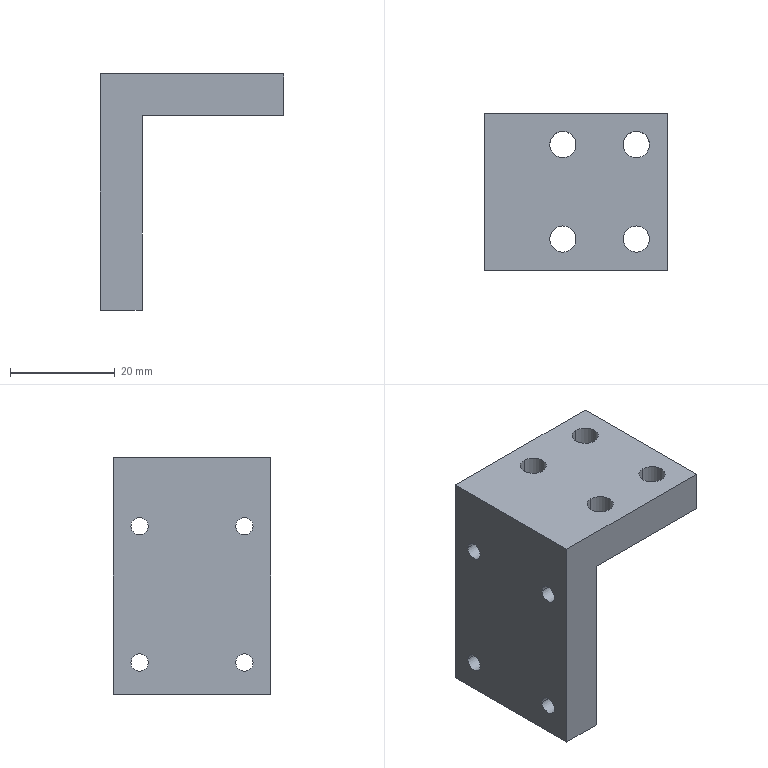Component | SolidWorks | DC-024-29-1 | 1 solid | 24 faces | box 35 x 30 x 45 mm | volume 16378 mm3 | cylinder 16 | plane 8 | commonest cylinder face diameters 3.3 x8 5 x8
build123d program:
from build123d import *

# Parameters (mm, degrees)
BOSS_EXTRUDE1_DEPTH = 15
M6_TAPPED_HOLE1_D   = 5
M4_TAPPED_HOLE1_D   = 3.3


with BuildPart() as part:
    # Sketch1 → Boss-Extrude1 (new, symmetric)
    with BuildSketch(Plane.XY):
        Polygon((-35, 0), (0, 0), (0, 45), (-8, 45), (-8, 8), (-35, 8), align=None)
    extrude(amount=BOSS_EXTRUDE1_DEPTH, both=True)

    # M6 Tapped Hole1 (through all)
    with Locations(Plane(origin=(0, 8, 0), x_dir=(1, 0, 0), z_dir=(0, 1, 0))):
        with Locations((-15, -9), (-15, 9), (-29, -9), (-29, 9)):
            Hole(M6_TAPPED_HOLE1_D / 2)

    # M4 Tapped Hole1 (through all)
    with Locations(Plane(origin=(0, 0, 0), x_dir=(0, 0, -1), z_dir=(1, 0, 0))):
        with Locations((10, 39), (-10, 39), (-10, 13), (10, 13)):
            Hole(M4_TAPPED_HOLE1_D / 2)


solid = part.part

# Placed as in the assembly
solid = solid.moved(Location((-61.333, 220.806, 63), (90, 0, -180)))
STEP:
#1=COLOUR_RGB('',0.7922,0.8196,0.9333);
#2=FILL_AREA_STYLE_COLOUR('',#1);
#3=FILL_AREA_STYLE('',(#2));
#4=SURFACE_STYLE_FILL_AREA(#3);
#5=SURFACE_SIDE_STYLE('',(#4));
#6=SURFACE_STYLE_USAGE(.BOTH.,#5);
#7=PRESENTATION_STYLE_ASSIGNMENT((#6));
#8=CARTESIAN_POINT('',(-2.1,9.022,0.9449));
#9=VERTEX_POINT('',#8);
#10=CARTESIAN_POINT('',(-2.1,9.152,0.9449));
#11=VERTEX_POINT('',#10);
#12=CARTESIAN_POINT('',(-2.1,9.087,0.9449));
#13=DIRECTION('',(-1.,0.,-0.));
#14=DIRECTION('',(0.,1.,0.));
#15=AXIS2_PLACEMENT_3D('',#12,#13,#14);
#16=CIRCLE('',#15,0.06496);
#17=EDGE_CURVE('',#9,#11,#16,.T.);
#18=ORIENTED_EDGE('',*,*,#17,.F.);
#19=CARTESIAN_POINT('',(-2.415,9.022,0.9449));
#20=VERTEX_POINT('',#19);
#21=CARTESIAN_POINT('',(-2.415,9.022,0.9449));
#22=DIRECTION('',(-1.,0.,-0.));
#23=VECTOR('',#22,39.37);
#24=LINE('',#21,#23);
#25=EDGE_CURVE('',#9,#20,#24,.T.);
#26=ORIENTED_EDGE('',*,*,#25,.T.);
#27=CARTESIAN_POINT('',(-2.415,9.152,0.9449));
#28=VERTEX_POINT('',#27);
#29=CARTESIAN_POINT('',(-2.415,9.087,0.9449));
#30=DIRECTION('',(-1.,0.,-0.));
#31=DIRECTION('',(0.,1.,0.));
#32=AXIS2_PLACEMENT_3D('',#29,#30,#31);
#33=CIRCLE('',#32,0.06496);
#34=EDGE_CURVE('',#20,#28,#33,.T.);
#35=ORIENTED_EDGE('',*,*,#34,.T.);
#36=CARTESIAN_POINT('',(-2.415,9.152,0.9449));
#37=DIRECTION('',(-1.,0.,-0.));
#38=VECTOR('',#37,39.37);
#39=LINE('',#36,#38);
#40=EDGE_CURVE('',#11,#28,#39,.T.);
#41=ORIENTED_EDGE('',*,*,#40,.F.);
#42=EDGE_LOOP('',(#18,#26,#35,#41));
#43=FACE_OUTER_BOUND('',#42,.T.);
#44=CARTESIAN_POINT('',(-2.415,9.087,0.9449));
#45=DIRECTION('',(-1.,0.,-0.));
#46=DIRECTION('',(0.,1.,0.));
#47=AXIS2_PLACEMENT_3D('',#44,#45,#46);
#48=CYLINDRICAL_SURFACE('',#47,0.06496);
#49=ADVANCED_FACE('',(#43),#48,.F.);
#50=CARTESIAN_POINT('',(-2.1,8.234,0.9449));
#51=VERTEX_POINT('',#50);
#52=CARTESIAN_POINT('',(-2.1,8.364,0.9449));
#53=VERTEX_POINT('',#52);
#54=CARTESIAN_POINT('',(-2.1,8.299,0.9449));
#55=DIRECTION('',(-1.,0.,-0.));
#56=DIRECTION('',(0.,1.,0.));
#57=AXIS2_PLACEMENT_3D('',#54,#55,#56);
#58=CIRCLE('',#57,0.06496);
#59=EDGE_CURVE('',#51,#53,#58,.T.);
#60=ORIENTED_EDGE('',*,*,#59,.F.);
#61=CARTESIAN_POINT('',(-2.415,8.234,0.9449));
#62=VERTEX_POINT('',#61);
#63=CARTESIAN_POINT('',(-2.415,8.234,0.9449));
#64=DIRECTION('',(-1.,0.,-0.));
#65=VECTOR('',#64,39.37);
#66=LINE('',#63,#65);
#67=EDGE_CURVE('',#51,#62,#66,.T.);
#68=ORIENTED_EDGE('',*,*,#67,.T.);
#69=CARTESIAN_POINT('',(-2.415,8.364,0.9449));
#70=VERTEX_POINT('',#69);
#71=CARTESIAN_POINT('',(-2.415,8.299,0.9449));
#72=DIRECTION('',(-1.,0.,-0.));
#73=DIRECTION('',(0.,1.,0.));
#74=AXIS2_PLACEMENT_3D('',#71,#72,#73);
#75=CIRCLE('',#74,0.06496);
#76=EDGE_CURVE('',#62,#70,#75,.T.);
#77=ORIENTED_EDGE('',*,*,#76,.T.);
#78=CARTESIAN_POINT('',(-2.415,8.364,0.9449));
#79=DIRECTION('',(-1.,0.,-0.));
#80=VECTOR('',#79,39.37);
#81=LINE('',#78,#80);
#82=EDGE_CURVE('',#53,#70,#81,.T.);
#83=ORIENTED_EDGE('',*,*,#82,.F.);
#84=EDGE_LOOP('',(#60,#68,#77,#83));
#85=FACE_OUTER_BOUND('',#84,.T.);
#86=CARTESIAN_POINT('',(-2.415,8.299,0.9449));
#87=DIRECTION('',(-1.,0.,-0.));
#88=DIRECTION('',(0.,1.,0.));
#89=AXIS2_PLACEMENT_3D('',#86,#87,#88);
#90=CYLINDRICAL_SURFACE('',#89,0.06496);
#91=ADVANCED_FACE('',(#85),#90,.F.);
#92=CARTESIAN_POINT('',(-2.1,8.234,1.969));
#93=VERTEX_POINT('',#92);
#94=CARTESIAN_POINT('',(-2.1,8.364,1.969));
#95=VERTEX_POINT('',#94);
#96=CARTESIAN_POINT('',(-2.1,8.299,1.969));
#97=DIRECTION('',(-1.,0.,-0.));
#98=DIRECTION('',(0.,1.,0.));
#99=AXIS2_PLACEMENT_3D('',#96,#97,#98);
#100=CIRCLE('',#99,0.06496);
#101=EDGE_CURVE('',#93,#95,#100,.T.);
#102=ORIENTED_EDGE('',*,*,#101,.F.);
#103=CARTESIAN_POINT('',(-2.415,8.234,1.969));
#104=VERTEX_POINT('',#103);
#105=CARTESIAN_POINT('',(-2.415,8.234,1.969));
#106=DIRECTION('',(-1.,0.,-0.));
#107=VECTOR('',#106,39.37);
#108=LINE('',#105,#107);
#109=EDGE_CURVE('',#93,#104,#108,.T.);
#110=ORIENTED_EDGE('',*,*,#109,.T.);
#111=CARTESIAN_POINT('',(-2.415,8.364,1.969));
#112=VERTEX_POINT('',#111);
#113=CARTESIAN_POINT('',(-2.415,8.299,1.969));
#114=DIRECTION('',(-1.,0.,-0.));
#115=DIRECTION('',(0.,1.,0.));
#116=AXIS2_PLACEMENT_3D('',#113,#114,#115);
#117=CIRCLE('',#116,0.06496);
#118=EDGE_CURVE('',#104,#112,#117,.T.);
#119=ORIENTED_EDGE('',*,*,#118,.T.);
#120=CARTESIAN_POINT('',(-2.415,8.364,1.969));
#121=DIRECTION('',(-1.,0.,-0.));
#122=VECTOR('',#121,39.37);
#123=LINE('',#120,#122);
#124=EDGE_CURVE('',#95,#112,#123,.T.);
#125=ORIENTED_EDGE('',*,*,#124,.F.);
#126=EDGE_LOOP('',(#102,#110,#119,#125));
#127=FACE_OUTER_BOUND('',#126,.T.);
#128=CARTESIAN_POINT('',(-2.415,8.299,1.969));
#129=DIRECTION('',(-1.,0.,-0.));
#130=DIRECTION('',(0.,1.,0.));
#131=AXIS2_PLACEMENT_3D('',#128,#129,#130);
#132=CYLINDRICAL_SURFACE('',#131,0.06496);
#133=ADVANCED_FACE('',(#127),#132,.F.);
#134=CARTESIAN_POINT('',(-2.1,9.022,1.969));
#135=VERTEX_POINT('',#134);
#136=CARTESIAN_POINT('',(-2.1,9.152,1.969));
#137=VERTEX_POINT('',#136);
#138=CARTESIAN_POINT('',(-2.1,9.087,1.969));
#139=DIRECTION('',(-1.,0.,-0.));
#140=DIRECTION('',(0.,1.,0.));
#141=AXIS2_PLACEMENT_3D('',#138,#139,#140);
#142=CIRCLE('',#141,0.06496);
#143=EDGE_CURVE('',#135,#137,#142,.T.);
#144=ORIENTED_EDGE('',*,*,#143,.F.);
#145=CARTESIAN_POINT('',(-2.415,9.022,1.969));
#146=VERTEX_POINT('',#145);
#147=CARTESIAN_POINT('',(-2.415,9.022,1.969));
#148=DIRECTION('',(-1.,0.,-0.));
#149=VECTOR('',#148,39.37);
#150=LINE('',#147,#149);
#151=EDGE_CURVE('',#135,#146,#150,.T.);
#152=ORIENTED_EDGE('',*,*,#151,.T.);
#153=CARTESIAN_POINT('',(-2.415,9.152,1.969));
#154=VERTEX_POINT('',#153);
#155=CARTESIAN_POINT('',(-2.415,9.087,1.969));
#156=DIRECTION('',(-1.,0.,-0.));
#157=DIRECTION('',(0.,1.,0.));
#158=AXIS2_PLACEMENT_3D('',#155,#156,#157);
#159=CIRCLE('',#158,0.06496);
#160=EDGE_CURVE('',#146,#154,#159,.T.);
#161=ORIENTED_EDGE('',*,*,#160,.T.);
#162=CARTESIAN_POINT('',(-2.415,9.152,1.969));
#163=DIRECTION('',(-1.,0.,-0.));
#164=VECTOR('',#163,39.37);
#165=LINE('',#162,#164);
#166=EDGE_CURVE('',#137,#154,#165,.T.);
#167=ORIENTED_EDGE('',*,*,#166,.F.);
#168=EDGE_LOOP('',(#144,#152,#161,#167));
#169=FACE_OUTER_BOUND('',#168,.T.);
#170=CARTESIAN_POINT('',(-2.415,9.087,1.969));
#171=DIRECTION('',(-1.,0.,-0.));
#172=DIRECTION('',(0.,1.,0.));
#173=AXIS2_PLACEMENT_3D('',#170,#171,#172);
#174=CYLINDRICAL_SURFACE('',#173,0.06496);
#175=ADVANCED_FACE('',(#169),#174,.F.);
#176=CARTESIAN_POINT('',(-1.824,8.437,2.48));
#177=VERTEX_POINT('',#176);
#178=CARTESIAN_POINT('',(-1.824,8.24,2.48));
#179=VERTEX_POINT('',#178);
#180=CARTESIAN_POINT('',(-1.824,8.339,2.48));
#181=DIRECTION('',(0.,-0.,-1.));
#182=DIRECTION('',(0.,-1.,0.));
#183=AXIS2_PLACEMENT_3D('',#180,#181,#182);
#184=CIRCLE('',#183,0.09843);
#185=EDGE_CURVE('',#177,#179,#184,.T.);
#186=ORIENTED_EDGE('',*,*,#185,.F.);
#187=CARTESIAN_POINT('',(-1.824,8.437,2.165));
#188=VERTEX_POINT('',#187);
#189=CARTESIAN_POINT('',(-1.824,8.437,2.165));
#190=DIRECTION('',(0.,-0.,-1.));
#191=VECTOR('',#190,39.37);
#192=LINE('',#189,#191);
#193=EDGE_CURVE('',#177,#188,#192,.T.);
#194=ORIENTED_EDGE('',*,*,#193,.T.);
#195=CARTESIAN_POINT('',(-1.824,8.24,2.165));
#196=VERTEX_POINT('',#195);
#197=CARTESIAN_POINT('',(-1.824,8.339,2.165));
#198=DIRECTION('',(0.,-0.,-1.));
#199=DIRECTION('',(0.,-1.,0.));
#200=AXIS2_PLACEMENT_3D('',#197,#198,#199);
#201=CIRCLE('',#200,0.09843);
#202=EDGE_CURVE('',#188,#196,#201,.T.);
#203=ORIENTED_EDGE('',*,*,#202,.T.);
#204=CARTESIAN_POINT('',(-1.824,8.24,2.165));
#205=DIRECTION('',(0.,-0.,-1.));
#206=VECTOR('',#205,39.37);
#207=LINE('',#204,#206);
#208=EDGE_CURVE('',#179,#196,#207,.T.);
#209=ORIENTED_EDGE('',*,*,#208,.F.);
#210=EDGE_LOOP('',(#186,#194,#203,#209));
#211=FACE_OUTER_BOUND('',#210,.T.);
#212=CARTESIAN_POINT('',(-1.824,8.339,2.165));
#213=DIRECTION('',(0.,-0.,-1.));
#214=DIRECTION('',(0.,-1.,0.));
#215=AXIS2_PLACEMENT_3D('',#212,#213,#214);
#216=CYLINDRICAL_SURFACE('',#215,0.09843);
#217=ADVANCED_FACE('',(#211),#216,.F.);
#218=CARTESIAN_POINT('',(-1.824,9.146,2.48));
#219=VERTEX_POINT('',#218);
#220=CARTESIAN_POINT('',(-1.824,8.949,2.48));
#221=VERTEX_POINT('',#220);
#222=CARTESIAN_POINT('',(-1.824,9.047,2.48));
#223=DIRECTION('',(0.,-0.,-1.));
#224=DIRECTION('',(0.,-1.,0.));
#225=AXIS2_PLACEMENT_3D('',#222,#223,#224);
#226=CIRCLE('',#225,0.09843);
#227=EDGE_CURVE('',#219,#221,#226,.T.);
#228=ORIENTED_EDGE('',*,*,#227,.F.);
#229=CARTESIAN_POINT('',(-1.824,9.146,2.165));
#230=VERTEX_POINT('',#229);
#231=CARTESIAN_POINT('',(-1.824,9.146,2.165));
#232=DIRECTION('',(0.,-0.,-1.));
#233=VECTOR('',#232,39.37);
#234=LINE('',#231,#233);
#235=EDGE_CURVE('',#219,#230,#234,.T.);
#236=ORIENTED_EDGE('',*,*,#235,.T.);
#237=CARTESIAN_POINT('',(-1.824,8.949,2.165));
#238=VERTEX_POINT('',#237);
#239=CARTESIAN_POINT('',(-1.824,9.047,2.165));
#240=DIRECTION('',(0.,-0.,-1.));
#241=DIRECTION('',(0.,-1.,0.));
#242=AXIS2_PLACEMENT_3D('',#239,#240,#241);
#243=CIRCLE('',#242,0.09843);
#244=EDGE_CURVE('',#230,#238,#243,.T.);
#245=ORIENTED_EDGE('',*,*,#244,.T.);
#246=CARTESIAN_POINT('',(-1.824,8.949,2.165));
#247=DIRECTION('',(0.,-0.,-1.));
#248=VECTOR('',#247,39.37);
#249=LINE('',#246,#248);
#250=EDGE_CURVE('',#221,#238,#249,.T.);
#251=ORIENTED_EDGE('',*,*,#250,.F.);
#252=EDGE_LOOP('',(#228,#236,#245,#251));
#253=FACE_OUTER_BOUND('',#252,.T.);
#254=CARTESIAN_POINT('',(-1.824,9.047,2.165));
#255=DIRECTION('',(0.,-0.,-1.));
#256=DIRECTION('',(0.,-1.,0.));
#257=AXIS2_PLACEMENT_3D('',#254,#255,#256);
#258=CYLINDRICAL_SURFACE('',#257,0.09843);
#259=ADVANCED_FACE('',(#253),#258,.F.);
#260=CARTESIAN_POINT('',(-1.273,8.437,2.48));
#261=VERTEX_POINT('',#260);
#262=CARTESIAN_POINT('',(-1.273,8.24,2.48));
#263=VERTEX_POINT('',#262);
#264=CARTESIAN_POINT('',(-1.273,8.339,2.48));
#265=DIRECTION('',(0.,-0.,-1.));
#266=DIRECTION('',(0.,-1.,0.));
#267=AXIS2_PLACEMENT_3D('',#264,#265,#266);
#268=CIRCLE('',#267,0.09843);
#269=EDGE_CURVE('',#261,#263,#268,.T.);
#270=ORIENTED_EDGE('',*,*,#269,.F.);
#271=CARTESIAN_POINT('',(-1.273,8.437,2.165));
#272=VERTEX_POINT('',#271);
#273=CARTESIAN_POINT('',(-1.273,8.437,2.165));
#274=DIRECTION('',(0.,-0.,-1.));
#275=VECTOR('',#274,39.37);
#276=LINE('',#273,#275);
#277=EDGE_CURVE('',#261,#272,#276,.T.);
#278=ORIENTED_EDGE('',*,*,#277,.T.);
#279=CARTESIAN_POINT('',(-1.273,8.24,2.165));
#280=VERTEX_POINT('',#279);
#281=CARTESIAN_POINT('',(-1.273,8.339,2.165));
#282=DIRECTION('',(0.,-0.,-1.));
#283=DIRECTION('',(0.,-1.,0.));
#284=AXIS2_PLACEMENT_3D('',#281,#282,#283);
#285=CIRCLE('',#284,0.09843);
#286=EDGE_CURVE('',#272,#280,#285,.T.);
#287=ORIENTED_EDGE('',*,*,#286,.T.);
#288=CARTESIAN_POINT('',(-1.273,8.24,2.165));
#289=DIRECTION('',(0.,-0.,-1.));
#290=VECTOR('',#289,39.37);
#291=LINE('',#288,#290);
#292=EDGE_CURVE('',#263,#280,#291,.T.);
#293=ORIENTED_EDGE('',*,*,#292,.F.);
#294=EDGE_LOOP('',(#270,#278,#287,#293));
#295=FACE_OUTER_BOUND('',#294,.T.);
#296=CARTESIAN_POINT('',(-1.273,8.339,2.165));
#297=DIRECTION('',(0.,-0.,-1.));
#298=DIRECTION('',(0.,-1.,0.));
#299=AXIS2_PLACEMENT_3D('',#296,#297,#298);
#300=CYLINDRICAL_SURFACE('',#299,0.09843);
#301=ADVANCED_FACE('',(#295),#300,.F.);
#302=CARTESIAN_POINT('',(-1.273,9.146,2.48));
#303=VERTEX_POINT('',#302);
#304=CARTESIAN_POINT('',(-1.273,8.949,2.48));
#305=VERTEX_POINT('',#304);
#306=CARTESIAN_POINT('',(-1.273,9.047,2.48));
#307=DIRECTION('',(0.,-0.,-1.));
#308=DIRECTION('',(0.,-1.,0.));
#309=AXIS2_PLACEMENT_3D('',#306,#307,#308);
#310=CIRCLE('',#309,0.09843);
#311=EDGE_CURVE('',#303,#305,#310,.T.);
#312=ORIENTED_EDGE('',*,*,#311,.F.);
#313=CARTESIAN_POINT('',(-1.273,9.146,2.165));
#314=VERTEX_POINT('',#313);
#315=CARTESIAN_POINT('',(-1.273,9.146,2.165));
#316=DIRECTION('',(0.,-0.,-1.));
#317=VECTOR('',#316,39.37);
#318=LINE('',#315,#317);
#319=EDGE_CURVE('',#303,#314,#318,.T.);
#320=ORIENTED_EDGE('',*,*,#319,.T.);
#321=CARTESIAN_POINT('',(-1.273,8.949,2.165));
#322=VERTEX_POINT('',#321);
#323=CARTESIAN_POINT('',(-1.273,9.047,2.165));
#324=DIRECTION('',(0.,-0.,-1.));
#325=DIRECTION('',(0.,-1.,0.));
#326=AXIS2_PLACEMENT_3D('',#323,#324,#325);
#327=CIRCLE('',#326,0.09843);
#328=EDGE_CURVE('',#314,#322,#327,.T.);
#329=ORIENTED_EDGE('',*,*,#328,.T.);
#330=CARTESIAN_POINT('',(-1.273,8.949,2.165));
#331=DIRECTION('',(0.,-0.,-1.));
#332=VECTOR('',#331,39.37);
#333=LINE('',#330,#332);
#334=EDGE_CURVE('',#305,#322,#333,.T.);
#335=ORIENTED_EDGE('',*,*,#334,.F.);
#336=EDGE_LOOP('',(#312,#320,#329,#335));
#337=FACE_OUTER_BOUND('',#336,.T.);
#338=CARTESIAN_POINT('',(-1.273,9.047,2.165));
#339=DIRECTION('',(0.,-0.,-1.));
#340=DIRECTION('',(0.,-1.,0.));
#341=AXIS2_PLACEMENT_3D('',#338,#339,#340);
#342=CYLINDRICAL_SURFACE('',#341,0.09843);
#343=ADVANCED_FACE('',(#337),#342,.F.);
#344=CARTESIAN_POINT('',(-1.037,9.284,2.165));
#345=VERTEX_POINT('',#344);
#346=CARTESIAN_POINT('',(-1.037,9.284,2.48));
#347=VERTEX_POINT('',#346);
#348=CARTESIAN_POINT('',(-1.037,9.284,2.165));
#349=DIRECTION('',(-0.,0.,1.));
#350=VECTOR('',#349,39.37);
#351=LINE('',#348,#350);
#352=EDGE_CURVE('',#345,#347,#351,.T.);
#353=ORIENTED_EDGE('',*,*,#352,.T.);
#354=CARTESIAN_POINT('',(-1.037,8.103,2.48));
#355=VERTEX_POINT('',#354);
#356=CARTESIAN_POINT('',(-1.037,8.103,2.48));
#357=DIRECTION('',(0.,1.,-0.));
#358=VECTOR('',#357,39.37);
#359=LINE('',#356,#358);
#360=EDGE_CURVE('',#355,#347,#359,.T.);
#361=ORIENTED_EDGE('',*,*,#360,.F.);
#362=CARTESIAN_POINT('',(-1.037,8.103,2.165));
#363=VERTEX_POINT('',#362);
#364=CARTESIAN_POINT('',(-1.037,8.103,2.165));
#365=DIRECTION('',(-0.,0.,1.));
#366=VECTOR('',#365,39.37);
#367=LINE('',#364,#366);
#368=EDGE_CURVE('',#363,#355,#367,.T.);
#369=ORIENTED_EDGE('',*,*,#368,.F.);
#370=CARTESIAN_POINT('',(-1.037,8.103,2.165));
#371=DIRECTION('',(0.,1.,-0.));
#372=VECTOR('',#371,39.37);
#373=LINE('',#370,#372);
#374=EDGE_CURVE('',#363,#345,#373,.T.);
#375=ORIENTED_EDGE('',*,*,#374,.T.);
#376=EDGE_LOOP('',(#353,#361,#369,#375));
#377=FACE_OUTER_BOUND('',#376,.T.);
#378=CARTESIAN_POINT('',(-1.037,8.103,2.165));
#379=DIRECTION('',(-1.,0.,-0.));
#380=DIRECTION('',(0.,1.,-0.));
#381=AXIS2_PLACEMENT_3D('',#378,#379,#380);
#382=PLANE('',#381);
#383=ADVANCED_FACE('',(#377),#382,.F.);
#384=CARTESIAN_POINT('',(-1.824,8.339,2.48));
#385=DIRECTION('',(0.,-0.,-1.));
#386=DIRECTION('',(0.,-1.,0.));
#387=AXIS2_PLACEMENT_3D('',#384,#385,#386);
#388=CIRCLE('',#387,0.09843);
#389=EDGE_CURVE('',#179,#177,#388,.T.);
#390=ORIENTED_EDGE('',*,*,#389,.T.);
#391=ORIENTED_EDGE('',*,*,#185,.T.);
#392=EDGE_LOOP('',(#390,#391));
#393=FACE_BOUND('',#392,.T.);
#394=CARTESIAN_POINT('',(-1.824,9.047,2.48));
#395=DIRECTION('',(0.,-0.,-1.));
#396=DIRECTION('',(0.,-1.,0.));
#397=AXIS2_PLACEMENT_3D('',#394,#395,#396);
#398=CIRCLE('',#397,0.09843);
#399=EDGE_CURVE('',#221,#219,#398,.T.);
#400=ORIENTED_EDGE('',*,*,#399,.T.);
#401=ORIENTED_EDGE('',*,*,#227,.T.);
#402=EDGE_LOOP('',(#400,#401));
#403=FACE_BOUND('',#402,.T.);
#404=CARTESIAN_POINT('',(-1.273,8.339,2.48));
#405=DIRECTION('',(0.,-0.,-1.));
#406=DIRECTION('',(0.,-1.,0.));
#407=AXIS2_PLACEMENT_3D('',#404,#405,#406);
#408=CIRCLE('',#407,0.09843);
#409=EDGE_CURVE('',#263,#261,#408,.T.);
#410=ORIENTED_EDGE('',*,*,#409,.T.);
#411=ORIENTED_EDGE('',*,*,#269,.T.);
#412=EDGE_LOOP('',(#410,#411));
#413=FACE_BOUND('',#412,.T.);
#414=CARTESIAN_POINT('',(-1.273,9.047,2.48));
#415=DIRECTION('',(0.,-0.,-1.));
#416=DIRECTION('',(0.,-1.,0.));
#417=AXIS2_PLACEMENT_3D('',#414,#415,#416);
#418=CIRCLE('',#417,0.09843);
#419=EDGE_CURVE('',#305,#303,#418,.T.);
#420=ORIENTED_EDGE('',*,*,#419,.T.);
#421=ORIENTED_EDGE('',*,*,#311,.T.);
#422=EDGE_LOOP('',(#420,#421));
#423=FACE_BOUND('',#422,.T.);
#424=CARTESIAN_POINT('',(-2.415,9.284,2.48));
#425=VERTEX_POINT('',#424);
#426=CARTESIAN_POINT('',(-1.037,9.284,2.48));
#427=DIRECTION('',(-1.,0.,-0.));
#428=VECTOR('',#427,39.37);
#429=LINE('',#426,#428);
#430=EDGE_CURVE('',#347,#425,#429,.T.);
#431=ORIENTED_EDGE('',*,*,#430,.T.);
#432=CARTESIAN_POINT('',(-2.415,8.103,2.48));
#433=VERTEX_POINT('',#432);
#434=CARTESIAN_POINT('',(-2.415,8.103,2.48));
#435=DIRECTION('',(0.,1.,-0.));
#436=VECTOR('',#435,39.37);
#437=LINE('',#434,#436);
#438=EDGE_CURVE('',#433,#425,#437,.T.);
#439=ORIENTED_EDGE('',*,*,#438,.F.);
#440=CARTESIAN_POINT('',(-1.037,8.103,2.48));
#441=DIRECTION('',(-1.,0.,-0.));
#442=VECTOR('',#441,39.37);
#443=LINE('',#440,#442);
#444=EDGE_CURVE('',#355,#433,#443,.T.);
#445=ORIENTED_EDGE('',*,*,#444,.F.);
#446=ORIENTED_EDGE('',*,*,#360,.T.);
#447=EDGE_LOOP('',(#431,#439,#445,#446));
#448=FACE_OUTER_BOUND('',#447,.T.);
#449=CARTESIAN_POINT('',(-1.037,8.103,2.48));
#450=DIRECTION('',(0.,-0.,-1.));
#451=DIRECTION('',(-0.,-1.,0.));
#452=AXIS2_PLACEMENT_3D('',#449,#450,#451);
#453=PLANE('',#452);
#454=ADVANCED_FACE('',(#393,#403,#413,#423,#448),#453,.F.);
#455=CARTESIAN_POINT('',(-2.415,9.087,0.9449));
#456=DIRECTION('',(-1.,0.,-0.));
#457=DIRECTION('',(0.,1.,0.));
#458=AXIS2_PLACEMENT_3D('',#455,#456,#457);
#459=CIRCLE('',#458,0.06496);
#460=EDGE_CURVE('',#28,#20,#459,.T.);
#461=ORIENTED_EDGE('',*,*,#460,.F.);
#462=ORIENTED_EDGE('',*,*,#34,.F.);
#463=EDGE_LOOP('',(#461,#462));
#464=FACE_BOUND('',#463,.T.);
#465=CARTESIAN_POINT('',(-2.415,8.299,0.9449));
#466=DIRECTION('',(-1.,0.,-0.));
#467=DIRECTION('',(0.,1.,0.));
#468=AXIS2_PLACEMENT_3D('',#465,#466,#467);
#469=CIRCLE('',#468,0.06496);
#470=EDGE_CURVE('',#70,#62,#469,.T.);
#471=ORIENTED_EDGE('',*,*,#470,.F.);
#472=ORIENTED_EDGE('',*,*,#76,.F.);
#473=EDGE_LOOP('',(#471,#472));
#474=FACE_BOUND('',#473,.T.);
#475=CARTESIAN_POINT('',(-2.415,8.299,1.969));
#476=DIRECTION('',(-1.,0.,-0.));
#477=DIRECTION('',(0.,1.,0.));
#478=AXIS2_PLACEMENT_3D('',#475,#476,#477);
#479=CIRCLE('',#478,0.06496);
#480=EDGE_CURVE('',#112,#104,#479,.T.);
#481=ORIENTED_EDGE('',*,*,#480,.F.);
#482=ORIENTED_EDGE('',*,*,#118,.F.);
#483=EDGE_LOOP('',(#481,#482));
#484=FACE_BOUND('',#483,.T.);
#485=CARTESIAN_POINT('',(-2.415,9.087,1.969));
#486=DIRECTION('',(-1.,0.,-0.));
#487=DIRECTION('',(0.,1.,0.));
#488=AXIS2_PLACEMENT_3D('',#485,#486,#487);
#489=CIRCLE('',#488,0.06496);
#490=EDGE_CURVE('',#154,#146,#489,.T.);
#491=ORIENTED_EDGE('',*,*,#490,.F.);
#492=ORIENTED_EDGE('',*,*,#160,.F.);
#493=EDGE_LOOP('',(#491,#492));
#494=FACE_BOUND('',#493,.T.);
#495=CARTESIAN_POINT('',(-2.415,9.284,0.7087));
#496=VERTEX_POINT('',#495);
#497=CARTESIAN_POINT('',(-2.415,9.284,2.48));
#498=DIRECTION('',(0.,-0.,-1.));
#499=VECTOR('',#498,39.37);
#500=LINE('',#497,#499);
#501=EDGE_CURVE('',#425,#496,#500,.T.);
#502=ORIENTED_EDGE('',*,*,#501,.T.);
#503=CARTESIAN_POINT('',(-2.415,8.103,0.7087));
#504=VERTEX_POINT('',#503);
#505=CARTESIAN_POINT('',(-2.415,8.103,0.7087));
#506=DIRECTION('',(0.,1.,-0.));
#507=VECTOR('',#506,39.37);
#508=LINE('',#505,#507);
#509=EDGE_CURVE('',#504,#496,#508,.T.);
#510=ORIENTED_EDGE('',*,*,#509,.F.);
#511=CARTESIAN_POINT('',(-2.415,8.103,2.48));
#512=DIRECTION('',(0.,-0.,-1.));
#513=VECTOR('',#512,39.37);
#514=LINE('',#511,#513);
#515=EDGE_CURVE('',#433,#504,#514,.T.);
#516=ORIENTED_EDGE('',*,*,#515,.F.);
#517=ORIENTED_EDGE('',*,*,#438,.T.);
#518=EDGE_LOOP('',(#502,#510,#516,#517));
#519=FACE_OUTER_BOUND('',#518,.T.);
#520=CARTESIAN_POINT('',(-2.415,8.103,2.48));
#521=DIRECTION('',(1.,-0.,0.));
#522=DIRECTION('',(-0.,-1.,0.));
#523=AXIS2_PLACEMENT_3D('',#520,#521,#522);
#524=PLANE('',#523);
#525=ADVANCED_FACE('',(#464,#474,#484,#494,#519),#524,.F.);
#526=CARTESIAN_POINT('',(-2.1,9.284,0.7087));
#527=VERTEX_POINT('',#526);
#528=CARTESIAN_POINT('',(-2.1,9.284,0.7087));
#529=DIRECTION('',(1.,-0.,0.));
#530=VECTOR('',#529,39.37);
#531=LINE('',#528,#530);
#532=EDGE_CURVE('',#496,#527,#531,.T.);
#533=ORIENTED_EDGE('',*,*,#532,.T.);
#534=CARTESIAN_POINT('',(-2.1,8.103,0.7087));
#535=VERTEX_POINT('',#534);
#536=CARTESIAN_POINT('',(-2.1,8.103,0.7087));
#537=DIRECTION('',(0.,1.,-0.));
#538=VECTOR('',#537,39.37);
#539=LINE('',#536,#538);
#540=EDGE_CURVE('',#535,#527,#539,.T.);
#541=ORIENTED_EDGE('',*,*,#540,.F.);
#542=CARTESIAN_POINT('',(-2.1,8.103,0.7087));
#543=DIRECTION('',(1.,-0.,0.));
#544=VECTOR('',#543,39.37);
#545=LINE('',#542,#544);
#546=EDGE_CURVE('',#504,#535,#545,.T.);
#547=ORIENTED_EDGE('',*,*,#546,.F.);
#548=ORIENTED_EDGE('',*,*,#509,.T.);
#549=EDGE_LOOP('',(#533,#541,#547,#548));
#550=FACE_OUTER_BOUND('',#549,.T.);
#551=CARTESIAN_POINT('',(-2.1,8.103,0.7087));
#552=DIRECTION('',(-0.,0.,1.));
#553=DIRECTION('',(0.,1.,-0.));
#554=AXIS2_PLACEMENT_3D('',#551,#552,#553);
#555=PLANE('',#554);
#556=ADVANCED_FACE('',(#550),#555,.F.);
#557=CARTESIAN_POINT('',(-2.1,9.087,0.9449));
#558=DIRECTION('',(-1.,0.,-0.));
#559=DIRECTION('',(0.,1.,0.));
#560=AXIS2_PLACEMENT_3D('',#557,#558,#559);
#561=CIRCLE('',#560,0.06496);
#562=EDGE_CURVE('',#11,#9,#561,.T.);
#563=ORIENTED_EDGE('',*,*,#562,.T.);
#564=ORIENTED_EDGE('',*,*,#17,.T.);
#565=EDGE_LOOP('',(#563,#564));
#566=FACE_BOUND('',#565,.T.);
#567=CARTESIAN_POINT('',(-2.1,8.299,0.9449));
#568=DIRECTION('',(-1.,0.,-0.));
#569=DIRECTION('',(0.,1.,0.));
#570=AXIS2_PLACEMENT_3D('',#567,#568,#569);
#571=CIRCLE('',#570,0.06496);
#572=EDGE_CURVE('',#53,#51,#571,.T.);
#573=ORIENTED_EDGE('',*,*,#572,.T.);
#574=ORIENTED_EDGE('',*,*,#59,.T.);
#575=EDGE_LOOP('',(#573,#574));
#576=FACE_BOUND('',#575,.T.);
#577=CARTESIAN_POINT('',(-2.1,8.299,1.969));
#578=DIRECTION('',(-1.,0.,-0.));
#579=DIRECTION('',(0.,1.,0.));
#580=AXIS2_PLACEMENT_3D('',#577,#578,#579);
#581=CIRCLE('',#580,0.06496);
#582=EDGE_CURVE('',#95,#93,#581,.T.);
#583=ORIENTED_EDGE('',*,*,#582,.T.);
#584=ORIENTED_EDGE('',*,*,#101,.T.);
#585=EDGE_LOOP('',(#583,#584));
#586=FACE_BOUND('',#585,.T.);
#587=CARTESIAN_POINT('',(-2.1,9.087,1.969));
#588=DIRECTION('',(-1.,0.,-0.));
#589=DIRECTION('',(0.,1.,0.));
#590=AXIS2_PLACEMENT_3D('',#587,#588,#589);
#591=CIRCLE('',#590,0.06496);
#592=EDGE_CURVE('',#137,#135,#591,.T.);
#593=ORIENTED_EDGE('',*,*,#592,.T.);
#594=ORIENTED_EDGE('',*,*,#143,.T.);
#595=EDGE_LOOP('',(#593,#594));
#596=FACE_BOUND('',#595,.T.);
#597=CARTESIAN_POINT('',(-2.1,9.284,2.165));
#598=VERTEX_POINT('',#597);
#599=CARTESIAN_POINT('',(-2.1,9.284,2.165));
#600=DIRECTION('',(-0.,0.,1.));
#601=VECTOR('',#600,39.37);
#602=LINE('',#599,#601);
#603=EDGE_CURVE('',#527,#598,#602,.T.);
#604=ORIENTED_EDGE('',*,*,#603,.T.);
#605=CARTESIAN_POINT('',(-2.1,8.103,2.165));
#606=VERTEX_POINT('',#605);
#607=CARTESIAN_POINT('',(-2.1,8.103,2.165));
#608=DIRECTION('',(0.,1.,-0.));
#609=VECTOR('',#608,39.37);
#610=LINE('',#607,#609);
#611=EDGE_CURVE('',#606,#598,#610,.T.);
#612=ORIENTED_EDGE('',*,*,#611,.F.);
#613=CARTESIAN_POINT('',(-2.1,8.103,2.165));
#614=DIRECTION('',(-0.,0.,1.));
#615=VECTOR('',#614,39.37);
#616=LINE('',#613,#615);
#617=EDGE_CURVE('',#535,#606,#616,.T.);
#618=ORIENTED_EDGE('',*,*,#617,.F.);
#619=ORIENTED_EDGE('',*,*,#540,.T.);
#620=EDGE_LOOP('',(#604,#612,#618,#619));
#621=FACE_OUTER_BOUND('',#620,.T.);
#622=CARTESIAN_POINT('',(-2.1,8.103,2.165));
#623=DIRECTION('',(-1.,0.,-0.));
#624=DIRECTION('',(0.,1.,-0.));
#625=AXIS2_PLACEMENT_3D('',#622,#623,#624);
#626=PLANE('',#625);
#627=ADVANCED_FACE('',(#566,#576,#586,#596,#621),#626,.F.);
#628=CARTESIAN_POINT('',(-1.824,8.339,2.165));
#629=DIRECTION('',(0.,-0.,-1.));
#630=DIRECTION('',(0.,-1.,0.));
#631=AXIS2_PLACEMENT_3D('',#628,#629,#630);
#632=CIRCLE('',#631,0.09843);
#633=EDGE_CURVE('',#196,#188,#632,.T.);
#634=ORIENTED_EDGE('',*,*,#633,.F.);
#635=ORIENTED_EDGE('',*,*,#202,.F.);
#636=EDGE_LOOP('',(#634,#635));
#637=FACE_BOUND('',#636,.T.);
#638=CARTESIAN_POINT('',(-1.824,9.047,2.165));
#639=DIRECTION('',(0.,-0.,-1.));
#640=DIRECTION('',(0.,-1.,0.));
#641=AXIS2_PLACEMENT_3D('',#638,#639,#640);
#642=CIRCLE('',#641,0.09843);
#643=EDGE_CURVE('',#238,#230,#642,.T.);
#644=ORIENTED_EDGE('',*,*,#643,.F.);
#645=ORIENTED_EDGE('',*,*,#244,.F.);
#646=EDGE_LOOP('',(#644,#645));
#647=FACE_BOUND('',#646,.T.);
#648=CARTESIAN_POINT('',(-1.273,8.339,2.165));
#649=DIRECTION('',(0.,-0.,-1.));
#650=DIRECTION('',(0.,-1.,0.));
#651=AXIS2_PLACEMENT_3D('',#648,#649,#650);
#652=CIRCLE('',#651,0.09843);
#653=EDGE_CURVE('',#280,#272,#652,.T.);
#654=ORIENTED_EDGE('',*,*,#653,.F.);
#655=ORIENTED_EDGE('',*,*,#286,.F.);
#656=EDGE_LOOP('',(#654,#655));
#657=FACE_BOUND('',#656,.T.);
#658=CARTESIAN_POINT('',(-1.273,9.047,2.165));
#659=DIRECTION('',(0.,-0.,-1.));
#660=DIRECTION('',(0.,-1.,0.));
#661=AXIS2_PLACEMENT_3D('',#658,#659,#660);
#662=CIRCLE('',#661,0.09843);
#663=EDGE_CURVE('',#322,#314,#662,.T.);
#664=ORIENTED_EDGE('',*,*,#663,.F.);
#665=ORIENTED_EDGE('',*,*,#328,.F.);
#666=EDGE_LOOP('',(#664,#665));
#667=FACE_BOUND('',#666,.T.);
#668=CARTESIAN_POINT('',(-1.037,9.284,2.165));
#669=DIRECTION('',(1.,-0.,0.));
#670=VECTOR('',#669,39.37);
#671=LINE('',#668,#670);
#672=EDGE_CURVE('',#598,#345,#671,.T.);
#673=ORIENTED_EDGE('',*,*,#672,.T.);
#674=ORIENTED_EDGE('',*,*,#374,.F.);
#675=CARTESIAN_POINT('',(-1.037,8.103,2.165));
#676=DIRECTION('',(1.,-0.,0.));
#677=VECTOR('',#676,39.37);
#678=LINE('',#675,#677);
#679=EDGE_CURVE('',#606,#363,#678,.T.);
#680=ORIENTED_EDGE('',*,*,#679,.F.);
#681=ORIENTED_EDGE('',*,*,#611,.T.);
#682=EDGE_LOOP('',(#673,#674,#680,#681));
#683=FACE_OUTER_BOUND('',#682,.T.);
#684=CARTESIAN_POINT('',(-1.037,8.103,2.165));
#685=DIRECTION('',(-0.,0.,1.));
#686=DIRECTION('',(0.,1.,-0.));
#687=AXIS2_PLACEMENT_3D('',#684,#685,#686);
#688=PLANE('',#687);
#689=ADVANCED_FACE('',(#637,#647,#657,#667,#683),#688,.F.);
#690=ORIENTED_EDGE('',*,*,#368,.T.);
#691=ORIENTED_EDGE('',*,*,#444,.T.);
#692=ORIENTED_EDGE('',*,*,#515,.T.);
#693=ORIENTED_EDGE('',*,*,#546,.T.);
#694=ORIENTED_EDGE('',*,*,#617,.T.);
#695=ORIENTED_EDGE('',*,*,#679,.T.);
#696=EDGE_LOOP('',(#690,#691,#692,#693,#694,#695));
#697=FACE_OUTER_BOUND('',#696,.T.);
#698=CARTESIAN_POINT('',(-2.415,8.103,2.48));
#699=DIRECTION('',(-0.,-1.,0.));
#700=DIRECTION('',(-1.,0.,-0.));
#701=AXIS2_PLACEMENT_3D('',#698,#699,#700);
#702=PLANE('',#701);
#703=ADVANCED_FACE('',(#697),#702,.T.);
#704=ORIENTED_EDGE('',*,*,#352,.F.);
#705=ORIENTED_EDGE('',*,*,#672,.F.);
#706=ORIENTED_EDGE('',*,*,#603,.F.);
#707=ORIENTED_EDGE('',*,*,#532,.F.);
#708=ORIENTED_EDGE('',*,*,#501,.F.);
#709=ORIENTED_EDGE('',*,*,#430,.F.);
#710=EDGE_LOOP('',(#704,#705,#706,#707,#708,#709));
#711=FACE_OUTER_BOUND('',#710,.T.);
#712=CARTESIAN_POINT('',(-2.415,9.284,2.48));
#713=DIRECTION('',(-0.,-1.,0.));
#714=DIRECTION('',(-1.,0.,-0.));
#715=AXIS2_PLACEMENT_3D('',#712,#713,#714);
#716=PLANE('',#715);
#717=ADVANCED_FACE('',(#711),#716,.F.);
#718=ORIENTED_EDGE('',*,*,#319,.F.);
#719=ORIENTED_EDGE('',*,*,#419,.F.);
#720=ORIENTED_EDGE('',*,*,#334,.T.);
#721=ORIENTED_EDGE('',*,*,#663,.T.);
#722=EDGE_LOOP('',(#718,#719,#720,#721));
#723=FACE_OUTER_BOUND('',#722,.T.);
#724=CARTESIAN_POINT('',(-1.273,9.047,2.165));
#725=DIRECTION('',(0.,-0.,-1.));
#726=DIRECTION('',(0.,-1.,0.));
#727=AXIS2_PLACEMENT_3D('',#724,#725,#726);
#728=CYLINDRICAL_SURFACE('',#727,0.09843);
#729=ADVANCED_FACE('',(#723),#728,.F.);
#730=ORIENTED_EDGE('',*,*,#277,.F.);
#731=ORIENTED_EDGE('',*,*,#409,.F.);
#732=ORIENTED_EDGE('',*,*,#292,.T.);
#733=ORIENTED_EDGE('',*,*,#653,.T.);
#734=EDGE_LOOP('',(#730,#731,#732,#733));
#735=FACE_OUTER_BOUND('',#734,.T.);
#736=CARTESIAN_POINT('',(-1.273,8.339,2.165));
#737=DIRECTION('',(0.,-0.,-1.));
#738=DIRECTION('',(0.,-1.,0.));
#739=AXIS2_PLACEMENT_3D('',#736,#737,#738);
#740=CYLINDRICAL_SURFACE('',#739,0.09843);
#741=ADVANCED_FACE('',(#735),#740,.F.);
#742=ORIENTED_EDGE('',*,*,#235,.F.);
#743=ORIENTED_EDGE('',*,*,#399,.F.);
#744=ORIENTED_EDGE('',*,*,#250,.T.);
#745=ORIENTED_EDGE('',*,*,#643,.T.);
#746=EDGE_LOOP('',(#742,#743,#744,#745));
#747=FACE_OUTER_BOUND('',#746,.T.);
#748=CARTESIAN_POINT('',(-1.824,9.047,2.165));
#749=DIRECTION('',(0.,-0.,-1.));
#750=DIRECTION('',(0.,-1.,0.));
#751=AXIS2_PLACEMENT_3D('',#748,#749,#750);
#752=CYLINDRICAL_SURFACE('',#751,0.09843);
#753=ADVANCED_FACE('',(#747),#752,.F.);
#754=ORIENTED_EDGE('',*,*,#193,.F.);
#755=ORIENTED_EDGE('',*,*,#389,.F.);
#756=ORIENTED_EDGE('',*,*,#208,.T.);
#757=ORIENTED_EDGE('',*,*,#633,.T.);
#758=EDGE_LOOP('',(#754,#755,#756,#757));
#759=FACE_OUTER_BOUND('',#758,.T.);
#760=CARTESIAN_POINT('',(-1.824,8.339,2.165));
#761=DIRECTION('',(0.,-0.,-1.));
#762=DIRECTION('',(0.,-1.,0.));
#763=AXIS2_PLACEMENT_3D('',#760,#761,#762);
#764=CYLINDRICAL_SURFACE('',#763,0.09843);
#765=ADVANCED_FACE('',(#759),#764,.F.);
#766=ORIENTED_EDGE('',*,*,#151,.F.);
#767=ORIENTED_EDGE('',*,*,#592,.F.);
#768=ORIENTED_EDGE('',*,*,#166,.T.);
#769=ORIENTED_EDGE('',*,*,#490,.T.);
#770=EDGE_LOOP('',(#766,#767,#768,#769));
#771=FACE_OUTER_BOUND('',#770,.T.);
#772=CARTESIAN_POINT('',(-2.415,9.087,1.969));
#773=DIRECTION('',(-1.,0.,-0.));
#774=DIRECTION('',(0.,1.,0.));
#775=AXIS2_PLACEMENT_3D('',#772,#773,#774);
#776=CYLINDRICAL_SURFACE('',#775,0.06496);
#777=ADVANCED_FACE('',(#771),#776,.F.);
#778=ORIENTED_EDGE('',*,*,#109,.F.);
#779=ORIENTED_EDGE('',*,*,#582,.F.);
#780=ORIENTED_EDGE('',*,*,#124,.T.);
#781=ORIENTED_EDGE('',*,*,#480,.T.);
#782=EDGE_LOOP('',(#778,#779,#780,#781));
#783=FACE_OUTER_BOUND('',#782,.T.);
#784=CARTESIAN_POINT('',(-2.415,8.299,1.969));
#785=DIRECTION('',(-1.,0.,-0.));
#786=DIRECTION('',(0.,1.,0.));
#787=AXIS2_PLACEMENT_3D('',#784,#785,#786);
#788=CYLINDRICAL_SURFACE('',#787,0.06496);
#789=ADVANCED_FACE('',(#783),#788,.F.);
#790=ORIENTED_EDGE('',*,*,#67,.F.);
#791=ORIENTED_EDGE('',*,*,#572,.F.);
#792=ORIENTED_EDGE('',*,*,#82,.T.);
#793=ORIENTED_EDGE('',*,*,#470,.T.);
#794=EDGE_LOOP('',(#790,#791,#792,#793));
#795=FACE_OUTER_BOUND('',#794,.T.);
#796=CARTESIAN_POINT('',(-2.415,8.299,0.9449));
#797=DIRECTION('',(-1.,0.,-0.));
#798=DIRECTION('',(0.,1.,0.));
#799=AXIS2_PLACEMENT_3D('',#796,#797,#798);
#800=CYLINDRICAL_SURFACE('',#799,0.06496);
#801=ADVANCED_FACE('',(#795),#800,.F.);
#802=ORIENTED_EDGE('',*,*,#25,.F.);
#803=ORIENTED_EDGE('',*,*,#562,.F.);
#804=ORIENTED_EDGE('',*,*,#40,.T.);
#805=ORIENTED_EDGE('',*,*,#460,.T.);
#806=EDGE_LOOP('',(#802,#803,#804,#805));
#807=FACE_OUTER_BOUND('',#806,.T.);
#808=CARTESIAN_POINT('',(-2.415,9.087,0.9449));
#809=DIRECTION('',(-1.,0.,-0.));
#810=DIRECTION('',(0.,1.,0.));
#811=AXIS2_PLACEMENT_3D('',#808,#809,#810);
#812=CYLINDRICAL_SURFACE('',#811,0.06496);
#813=ADVANCED_FACE('',(#807),#812,.F.);
#814=CLOSED_SHELL('',(#49,#91,#133,#175,#217,#259,#301,#343,#383,#454,#525,#556,#627,#689,#703,#717,#729,#741,#753,#765,#777,#789,#801,#813));
#815=MANIFOLD_SOLID_BREP('',#814);
#816=STYLED_ITEM('',(#7),#815);
#817=(LENGTH_UNIT()NAMED_UNIT(*)SI_UNIT($,.METRE.));
#818=LENGTH_MEASURE_WITH_UNIT(LENGTH_MEASURE(0.0254),#817);
#819=DIMENSIONAL_EXPONENTS(1.,0.,0.,0.,0.,0.,0.);
#820=(CONVERSION_BASED_UNIT('',#818)LENGTH_UNIT()NAMED_UNIT(#819));
#821=UNCERTAINTY_MEASURE_WITH_UNIT(LENGTH_MEASURE(0.00001),#820,'','');
#822=(NAMED_UNIT(*)PLANE_ANGLE_UNIT()SI_UNIT($,.RADIAN.));
#823=(NAMED_UNIT(*)SI_UNIT($,.STERADIAN.)SOLID_ANGLE_UNIT());
#824=(GEOMETRIC_REPRESENTATION_CONTEXT(3)GLOBAL_UNCERTAINTY_ASSIGNED_CONTEXT((#821))GLOBAL_UNIT_ASSIGNED_CONTEXT((#820,#822,#823))REPRESENTATION_CONTEXT('',''));
#825=MECHANICAL_DESIGN_GEOMETRIC_PRESENTATION_REPRESENTATION('',(#816),#824);
#826=PRESENTATION_LAYER_ASSIGNMENT('','',(#816));
#827=CARTESIAN_POINT('',(0.,0.,0.));
#828=DIRECTION('',(0.,0.,1.));
#829=DIRECTION('',(1.,0.,0.));
#830=AXIS2_PLACEMENT_3D('',#827,#828,#829);
#831=(LENGTH_UNIT()NAMED_UNIT(*)SI_UNIT($,.METRE.));
#832=LENGTH_MEASURE_WITH_UNIT(LENGTH_MEASURE(0.0254),#831);
#833=DIMENSIONAL_EXPONENTS(1.,0.,0.,0.,0.,0.,0.);
#834=(CONVERSION_BASED_UNIT('',#832)LENGTH_UNIT()NAMED_UNIT(#833));
#835=UNCERTAINTY_MEASURE_WITH_UNIT(LENGTH_MEASURE(0.00001),#834,'','');
#836=(NAMED_UNIT(*)PLANE_ANGLE_UNIT()SI_UNIT($,.RADIAN.));
#837=(NAMED_UNIT(*)SI_UNIT($,.STERADIAN.)SOLID_ANGLE_UNIT());
#838=(GEOMETRIC_REPRESENTATION_CONTEXT(3)GLOBAL_UNCERTAINTY_ASSIGNED_CONTEXT((#835))GLOBAL_UNIT_ASSIGNED_CONTEXT((#834,#836,#837))REPRESENTATION_CONTEXT('',''));
#839=ADVANCED_BREP_SHAPE_REPRESENTATION('',(#815,#830),#838);